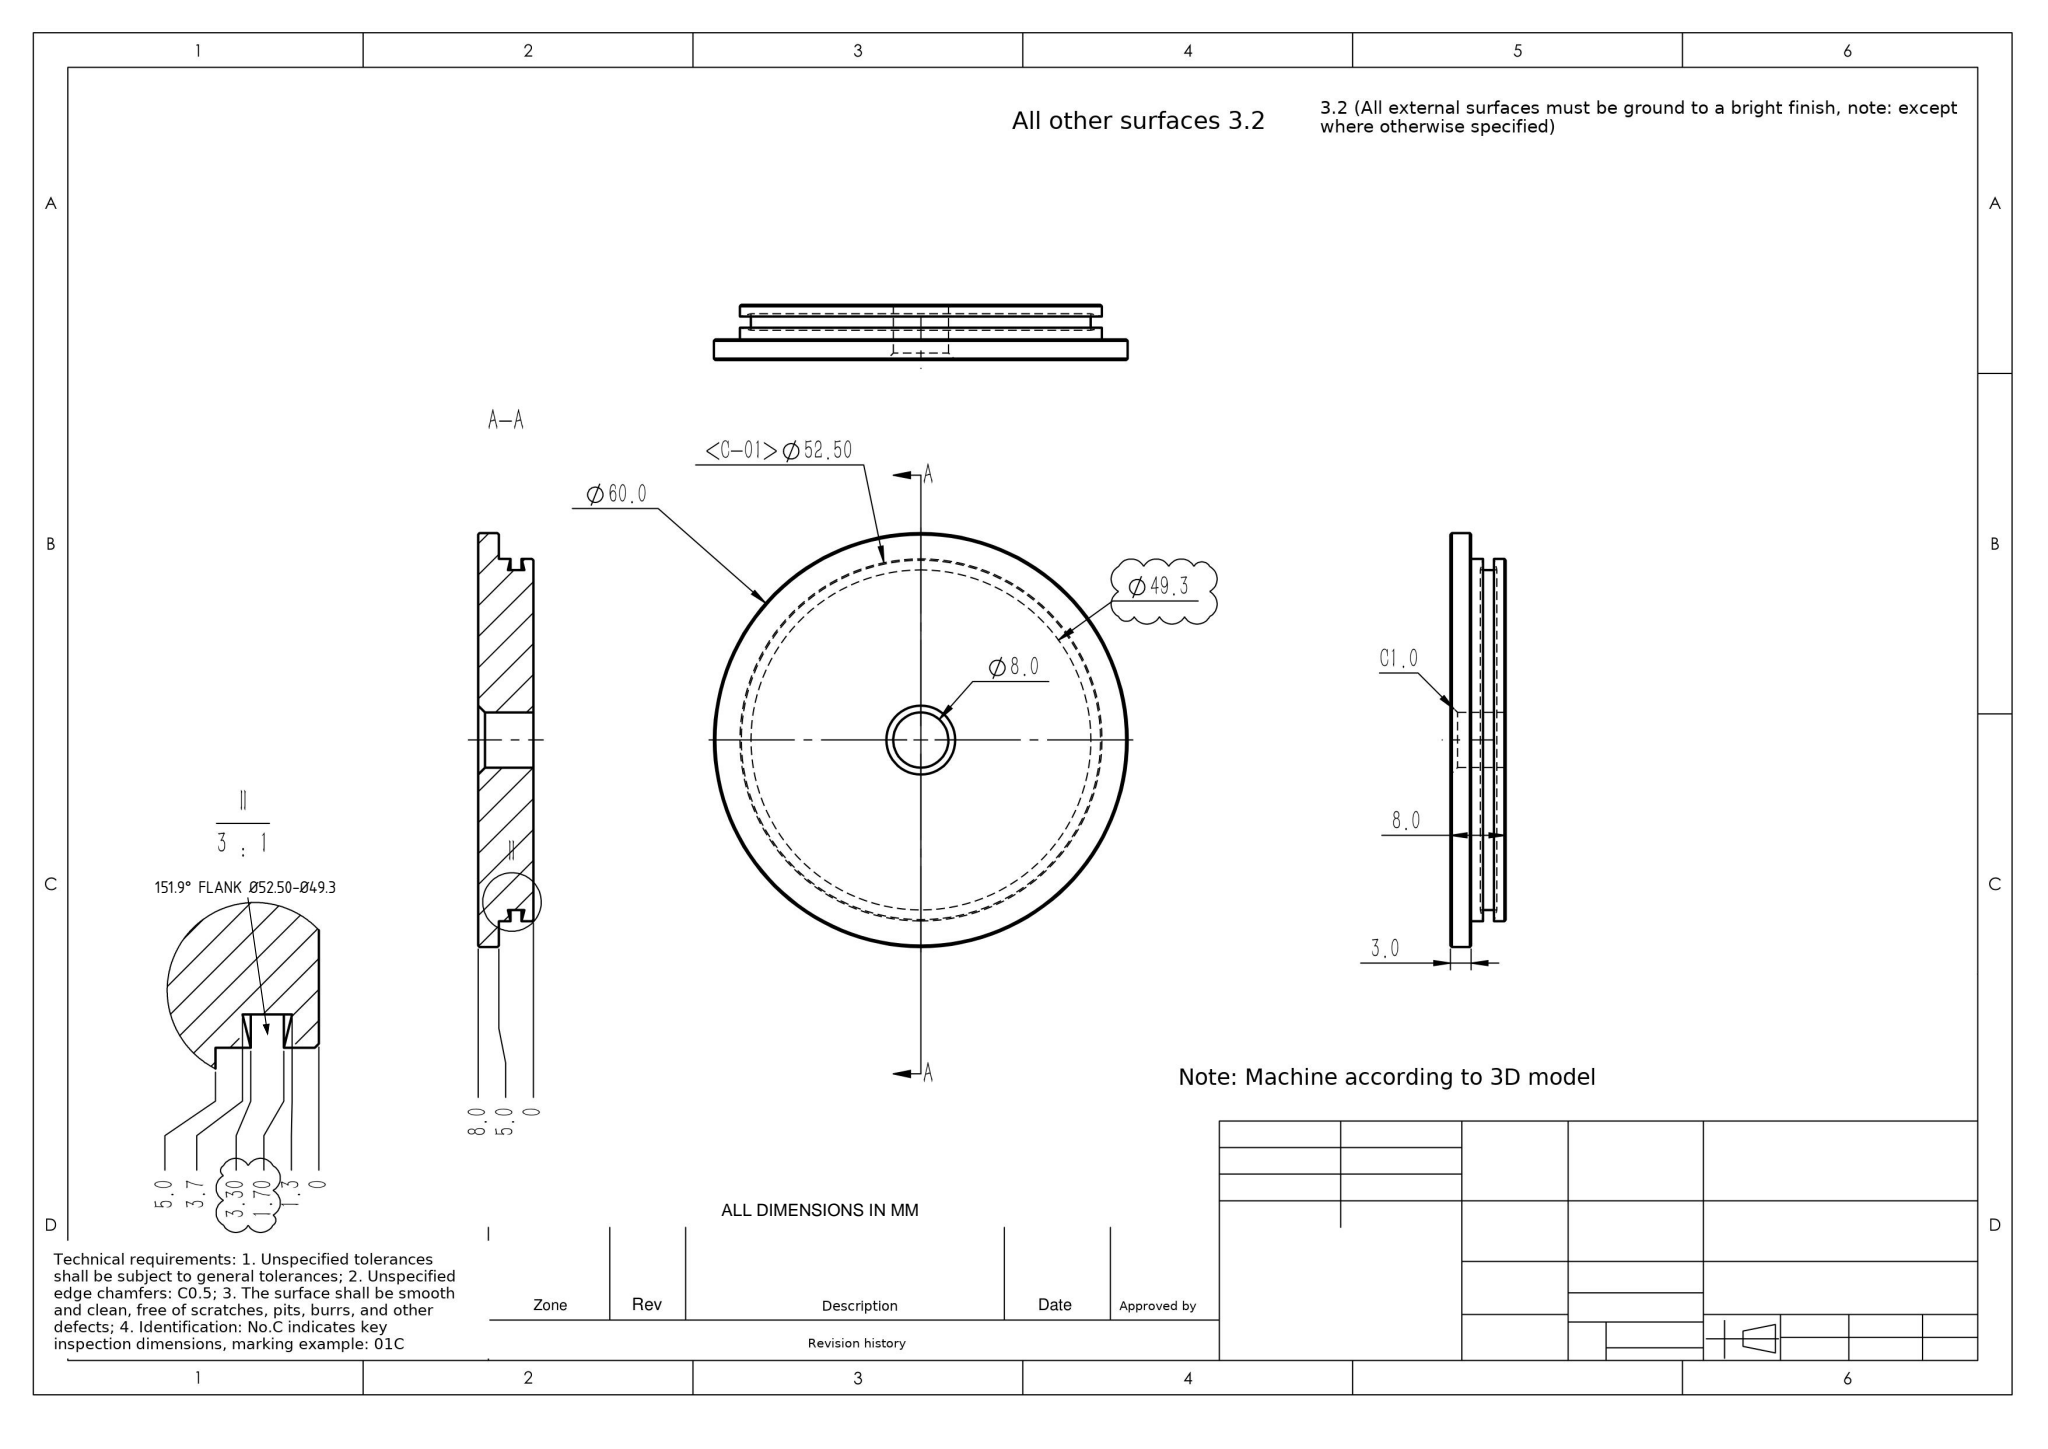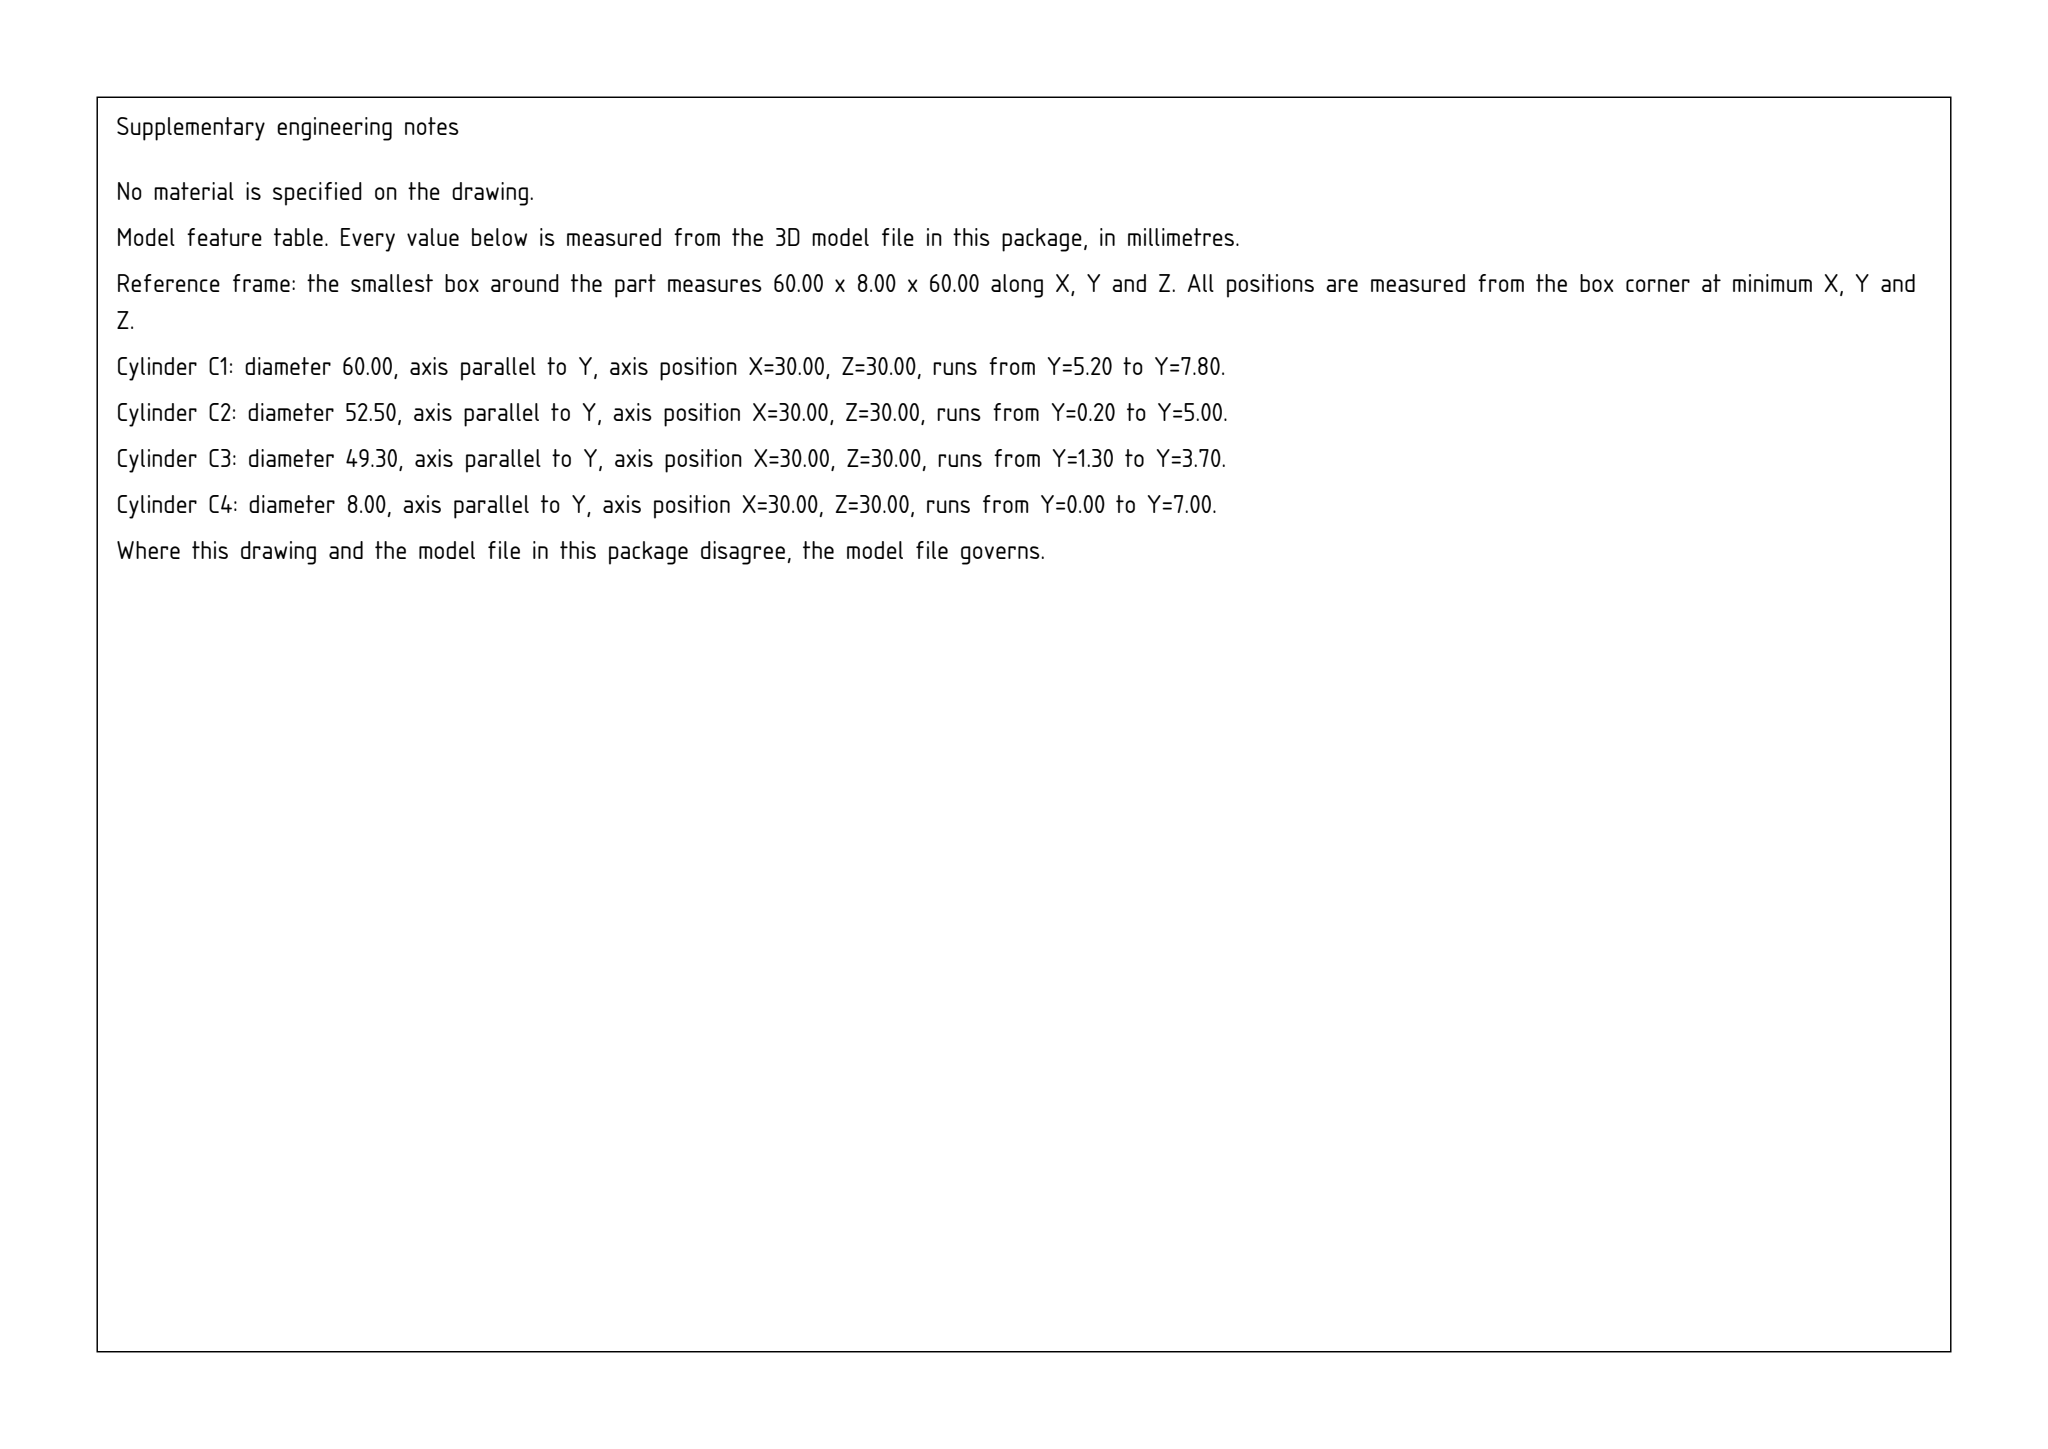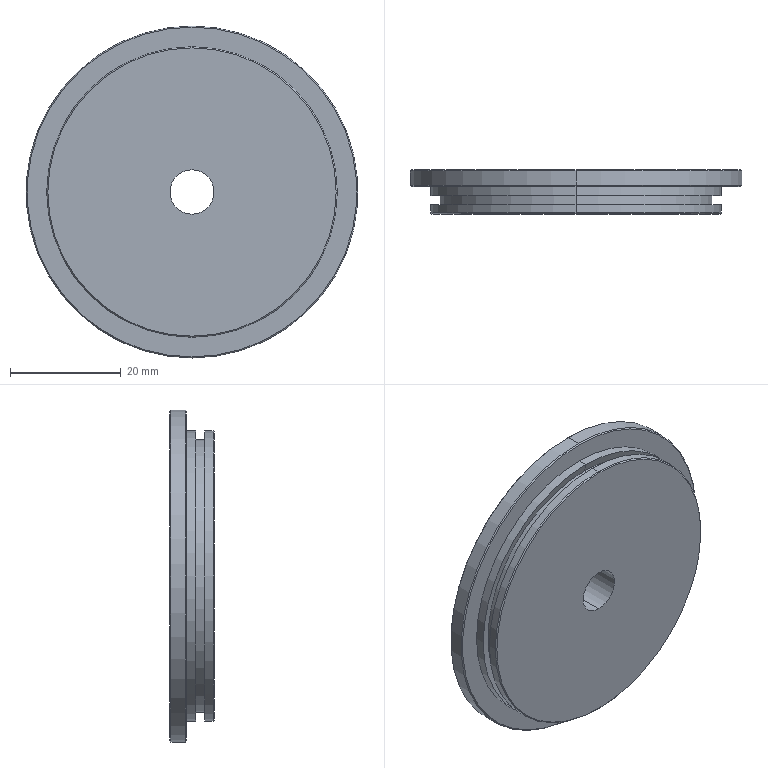Part | SolidWorks | mm | 1 solid | 25 faces | box 60 x 8 x 60 mm | volume 18369 mm3 | cone 12 | cylinder 10 | plane 3 | commonest cylinder face diameters 52.5 x4 49.3 x2 8 x2 60 x2
Drawing notes:
DETAIL II: GROOVE FLANK 151.9° INCL, Ø52.50 TO Ø49.3 | from the solid: cones[included_angle,ref_dia]: [151.9, 52.5] and [151.9, 49.3], both x2
build123d program:
from build123d import *

# Parameters (mm, degrees)
SKETCH1_R           = 30
BOSS_EXTRUDE1_DEPTH = 3
SKETCH2_R           = 4
CUT_EXTRUDE1_DEPTH  = 5
CHAMFER1_SIZE       = 1
SKETCH3_R           = 26.25
SKETCH3_R_2         = 4
BOSS_EXTRUDE2_DEPTH = 5
CHAMFER2_SIZE       = 0.2


with BuildPart() as part:
    # Sketch1 → Boss-Extrude1 (new body)
    with BuildSketch(Plane(origin=(0, 0, 0), x_dir=(1, 0, 0), z_dir=(0, 1, 0))):
        with Locations(Location((0, 0, 0), (0, 0, 270))):
            Circle(SKETCH1_R)
    extrude(amount=BOSS_EXTRUDE1_DEPTH)

    # Sketch2 → Cut-Extrude1 (cut)
    with BuildSketch(Plane(origin=(0, 3, 0), x_dir=(1, 0, 0), z_dir=(0, 1, 0))):
        with Locations(Location((0, 0, 0), (0, 0, 270))):
            Circle(SKETCH2_R)
    extrude(amount=-CUT_EXTRUDE1_DEPTH, mode=Mode.SUBTRACT)

    # Chamfer1
    chamfer1_edges = [part.edges().sort_by_distance(p)[0] for p in [
        (0, 3, -4),
    ]]
    chamfer(chamfer1_edges, length=CHAMFER1_SIZE)

    # Sketch3 → Boss-Extrude2 (add)
    with BuildSketch(Plane.XZ):
        with Locations(Location((0, 0, 0), (0, 0, 90))):
            Circle(SKETCH3_R)
        with Locations(Location((0, 0, 0), (0, 0, 90))):
            Circle(SKETCH3_R_2, mode=Mode.SUBTRACT)
    extrude(amount=BOSS_EXTRUDE2_DEPTH)

    # Sketch5 → Cut-Revolve1 (revolve, cut)
    with BuildSketch(Plane.XY, mode=Mode.PRIVATE) as cut_revolve1_sk:
        Polygon((-26.25, -1.7), (-26.25, -3.3), (-24.65, -3.7), (-24.65, -1.3), align=None)
    revolve(cut_revolve1_sk.sketch.rotate(Axis((0, -2, 0), (0, 1, 0)), 270), axis=Axis((0, -2, 0), (0, 1, 0)), mode=Mode.SUBTRACT)

    # Chamfer2
    chamfer2_edges = [part.edges().sort_by_distance(p)[0] for p in [
        (0, -5, -26.25),
        (0, 0, -30),
        (0, 3, -30),
    ]]
    chamfer(chamfer2_edges, length=CHAMFER2_SIZE)


solid = part.part
STEP:
#1=CARTESIAN_POINT('',(0.,-5.,-26.05));
#2=VERTEX_POINT('',#1);
#3=CARTESIAN_POINT('',(0.,-5.,26.05));
#4=VERTEX_POINT('',#3);
#5=CARTESIAN_POINT('',(0.,-5.,0.));
#6=DIRECTION('',(0.,-1.,0.));
#7=DIRECTION('',(0.,0.,-1.));
#8=AXIS2_PLACEMENT_3D('',#5,#6,#7);
#9=CIRCLE('',#8,26.05);
#10=EDGE_CURVE('',#2,#4,#9,.T.);
#11=ORIENTED_EDGE('',*,*,#10,.F.);
#12=CARTESIAN_POINT('',(0.,-4.8,-26.25));
#13=VERTEX_POINT('',#12);
#14=CARTESIAN_POINT('',(0.,-5.,-26.05));
#15=DIRECTION('',(0.,0.7071,-0.7071));
#16=VECTOR('',#15,1000.);
#17=LINE('',#14,#16);
#18=EDGE_CURVE('',#2,#13,#17,.T.);
#19=ORIENTED_EDGE('',*,*,#18,.T.);
#20=CARTESIAN_POINT('',(0.,-4.8,26.25));
#21=VERTEX_POINT('',#20);
#22=CARTESIAN_POINT('',(0.,-4.8,0.));
#23=DIRECTION('',(0.,1.,0.));
#24=DIRECTION('',(0.,0.,-1.));
#25=AXIS2_PLACEMENT_3D('',#22,#23,#24);
#26=CIRCLE('',#25,26.25);
#27=EDGE_CURVE('',#21,#13,#26,.T.);
#28=ORIENTED_EDGE('',*,*,#27,.F.);
#29=CARTESIAN_POINT('',(0.,-5.,26.05));
#30=DIRECTION('',(0.,0.7071,0.7071));
#31=VECTOR('',#30,1000.);
#32=LINE('',#29,#31);
#33=EDGE_CURVE('',#4,#21,#32,.T.);
#34=ORIENTED_EDGE('',*,*,#33,.F.);
#35=EDGE_LOOP('',(#11,#19,#28,#34));
#36=FACE_OUTER_BOUND('',#35,.T.);
#37=CARTESIAN_POINT('',(0.,-5.,0.));
#38=DIRECTION('',(0.,1.,0.));
#39=DIRECTION('',(0.,0.,1.));
#40=AXIS2_PLACEMENT_3D('',#37,#38,#39);
#41=CONICAL_SURFACE('',#40,26.05,0.7854);
#42=ADVANCED_FACE('',(#36),#41,.T.);
#43=CARTESIAN_POINT('',(0.,3.,29.8));
#44=VERTEX_POINT('',#43);
#45=CARTESIAN_POINT('',(0.,3.,-29.8));
#46=VERTEX_POINT('',#45);
#47=CARTESIAN_POINT('',(0.,3.,0.));
#48=DIRECTION('',(0.,1.,0.));
#49=DIRECTION('',(0.,0.,1.));
#50=AXIS2_PLACEMENT_3D('',#47,#48,#49);
#51=CIRCLE('',#50,29.8);
#52=EDGE_CURVE('',#44,#46,#51,.T.);
#53=ORIENTED_EDGE('',*,*,#52,.F.);
#54=CARTESIAN_POINT('',(0.,2.8,30.));
#55=VERTEX_POINT('',#54);
#56=CARTESIAN_POINT('',(0.,3.,29.8));
#57=DIRECTION('',(0.,-0.7071,0.7071));
#58=VECTOR('',#57,1000.);
#59=LINE('',#56,#58);
#60=EDGE_CURVE('',#44,#55,#59,.T.);
#61=ORIENTED_EDGE('',*,*,#60,.T.);
#62=CARTESIAN_POINT('',(0.,2.8,-30.));
#63=VERTEX_POINT('',#62);
#64=CARTESIAN_POINT('',(0.,2.8,0.));
#65=DIRECTION('',(0.,-1.,0.));
#66=DIRECTION('',(0.,0.,1.));
#67=AXIS2_PLACEMENT_3D('',#64,#65,#66);
#68=CIRCLE('',#67,30.);
#69=EDGE_CURVE('',#63,#55,#68,.T.);
#70=ORIENTED_EDGE('',*,*,#69,.F.);
#71=CARTESIAN_POINT('',(0.,3.,-29.8));
#72=DIRECTION('',(0.,-0.7071,-0.7071));
#73=VECTOR('',#72,1000.);
#74=LINE('',#71,#73);
#75=EDGE_CURVE('',#46,#63,#74,.T.);
#76=ORIENTED_EDGE('',*,*,#75,.F.);
#77=EDGE_LOOP('',(#53,#61,#70,#76));
#78=FACE_OUTER_BOUND('',#77,.T.);
#79=CARTESIAN_POINT('',(0.,3.,0.));
#80=DIRECTION('',(0.,-1.,0.));
#81=DIRECTION('',(0.,0.,-1.));
#82=AXIS2_PLACEMENT_3D('',#79,#80,#81);
#83=CONICAL_SURFACE('',#82,29.8,0.7854);
#84=ADVANCED_FACE('',(#78),#83,.T.);
#85=CARTESIAN_POINT('',(0.,0.,-29.8));
#86=VERTEX_POINT('',#85);
#87=CARTESIAN_POINT('',(0.,0.,29.8));
#88=VERTEX_POINT('',#87);
#89=CARTESIAN_POINT('',(0.,0.,0.));
#90=DIRECTION('',(0.,-1.,0.));
#91=DIRECTION('',(0.,0.,1.));
#92=AXIS2_PLACEMENT_3D('',#89,#90,#91);
#93=CIRCLE('',#92,29.8);
#94=EDGE_CURVE('',#86,#88,#93,.T.);
#95=ORIENTED_EDGE('',*,*,#94,.F.);
#96=CARTESIAN_POINT('',(0.,0.2,-30.));
#97=VERTEX_POINT('',#96);
#98=CARTESIAN_POINT('',(0.,0.2,-30.));
#99=DIRECTION('',(0.,0.7071,-0.7071));
#100=VECTOR('',#99,1000.);
#101=LINE('',#98,#100);
#102=EDGE_CURVE('',#86,#97,#101,.T.);
#103=ORIENTED_EDGE('',*,*,#102,.T.);
#104=CARTESIAN_POINT('',(0.,0.2,30.));
#105=VERTEX_POINT('',#104);
#106=CARTESIAN_POINT('',(0.,0.2,0.));
#107=DIRECTION('',(0.,1.,0.));
#108=DIRECTION('',(0.,0.,1.));
#109=AXIS2_PLACEMENT_3D('',#106,#107,#108);
#110=CIRCLE('',#109,30.);
#111=EDGE_CURVE('',#105,#97,#110,.T.);
#112=ORIENTED_EDGE('',*,*,#111,.F.);
#113=CARTESIAN_POINT('',(0.,0.2,30.));
#114=DIRECTION('',(0.,0.7071,0.7071));
#115=VECTOR('',#114,1000.);
#116=LINE('',#113,#115);
#117=EDGE_CURVE('',#88,#105,#116,.T.);
#118=ORIENTED_EDGE('',*,*,#117,.F.);
#119=EDGE_LOOP('',(#95,#103,#112,#118));
#120=FACE_OUTER_BOUND('',#119,.T.);
#121=CARTESIAN_POINT('',(0.,0.2,0.));
#122=DIRECTION('',(0.,1.,0.));
#123=DIRECTION('',(0.,0.,1.));
#124=AXIS2_PLACEMENT_3D('',#121,#122,#123);
#125=CONICAL_SURFACE('',#124,30.,0.7854);
#126=ADVANCED_FACE('',(#120),#125,.T.);
#127=CARTESIAN_POINT('',(0.,-3.7,24.65));
#128=VERTEX_POINT('',#127);
#129=CARTESIAN_POINT('',(0.,-3.7,-24.65));
#130=VERTEX_POINT('',#129);
#131=CARTESIAN_POINT('',(0.,-3.7,0.));
#132=DIRECTION('',(0.,-1.,0.));
#133=DIRECTION('',(0.,0.,-1.));
#134=AXIS2_PLACEMENT_3D('',#131,#132,#133);
#135=CIRCLE('',#134,24.65);
#136=EDGE_CURVE('',#128,#130,#135,.T.);
#137=ORIENTED_EDGE('',*,*,#136,.T.);
#138=CARTESIAN_POINT('',(0.,-3.3,-26.25));
#139=VERTEX_POINT('',#138);
#140=CARTESIAN_POINT('',(0.,-3.3,-26.25));
#141=DIRECTION('',(0.,0.2425,-0.9701));
#142=VECTOR('',#141,1000.);
#143=LINE('',#140,#142);
#144=EDGE_CURVE('',#130,#139,#143,.T.);
#145=ORIENTED_EDGE('',*,*,#144,.T.);
#146=CARTESIAN_POINT('',(0.,-3.3,26.25));
#147=VERTEX_POINT('',#146);
#148=CARTESIAN_POINT('',(0.,-3.3,0.));
#149=DIRECTION('',(0.,-1.,0.));
#150=DIRECTION('',(0.,0.,-1.));
#151=AXIS2_PLACEMENT_3D('',#148,#149,#150);
#152=CIRCLE('',#151,26.25);
#153=EDGE_CURVE('',#147,#139,#152,.T.);
#154=ORIENTED_EDGE('',*,*,#153,.F.);
#155=CARTESIAN_POINT('',(0.,-3.3,26.25));
#156=DIRECTION('',(0.,0.2425,0.9701));
#157=VECTOR('',#156,1000.);
#158=LINE('',#155,#157);
#159=EDGE_CURVE('',#128,#147,#158,.T.);
#160=ORIENTED_EDGE('',*,*,#159,.F.);
#161=EDGE_LOOP('',(#137,#145,#154,#160));
#162=FACE_OUTER_BOUND('',#161,.T.);
#163=CARTESIAN_POINT('',(0.,-3.3,0.));
#164=DIRECTION('',(0.,1.,0.));
#165=DIRECTION('',(0.,0.,1.));
#166=AXIS2_PLACEMENT_3D('',#163,#164,#165);
#167=CONICAL_SURFACE('',#166,26.25,1.326);
#168=ADVANCED_FACE('',(#162),#167,.F.);
#169=CARTESIAN_POINT('',(0.,-1.3,-24.65));
#170=VERTEX_POINT('',#169);
#171=CARTESIAN_POINT('',(0.,-1.3,24.65));
#172=VERTEX_POINT('',#171);
#173=CARTESIAN_POINT('',(0.,-1.3,0.));
#174=DIRECTION('',(0.,-1.,0.));
#175=DIRECTION('',(0.,0.,-1.));
#176=AXIS2_PLACEMENT_3D('',#173,#174,#175);
#177=CIRCLE('',#176,24.65);
#178=EDGE_CURVE('',#170,#172,#177,.T.);
#179=ORIENTED_EDGE('',*,*,#178,.T.);
#180=CARTESIAN_POINT('',(0.,-5.,24.65));
#181=DIRECTION('',(0.,-1.,0.));
#182=VECTOR('',#181,1000.);
#183=LINE('',#180,#182);
#184=EDGE_CURVE('',#172,#128,#183,.T.);
#185=ORIENTED_EDGE('',*,*,#184,.T.);
#186=CARTESIAN_POINT('',(0.,-3.7,0.));
#187=DIRECTION('',(0.,-1.,0.));
#188=DIRECTION('',(0.,0.,-1.));
#189=AXIS2_PLACEMENT_3D('',#186,#187,#188);
#190=CIRCLE('',#189,24.65);
#191=EDGE_CURVE('',#130,#128,#190,.T.);
#192=ORIENTED_EDGE('',*,*,#191,.F.);
#193=CARTESIAN_POINT('',(0.,-5.,-24.65));
#194=DIRECTION('',(0.,-1.,0.));
#195=VECTOR('',#194,1000.);
#196=LINE('',#193,#195);
#197=EDGE_CURVE('',#170,#130,#196,.T.);
#198=ORIENTED_EDGE('',*,*,#197,.F.);
#199=EDGE_LOOP('',(#179,#185,#192,#198));
#200=FACE_OUTER_BOUND('',#199,.T.);
#201=CARTESIAN_POINT('',(0.,-5.,0.));
#202=DIRECTION('',(0.,-1.,0.));
#203=DIRECTION('',(0.,0.,-1.));
#204=AXIS2_PLACEMENT_3D('',#201,#202,#203);
#205=CYLINDRICAL_SURFACE('',#204,24.65);
#206=ADVANCED_FACE('',(#200),#205,.T.);
#207=CARTESIAN_POINT('',(0.,-1.3,0.));
#208=DIRECTION('',(0.,-1.,0.));
#209=DIRECTION('',(0.,0.,-1.));
#210=AXIS2_PLACEMENT_3D('',#207,#208,#209);
#211=CIRCLE('',#210,24.65);
#212=EDGE_CURVE('',#172,#170,#211,.T.);
#213=ORIENTED_EDGE('',*,*,#212,.F.);
#214=CARTESIAN_POINT('',(0.,-1.7,26.25));
#215=VERTEX_POINT('',#214);
#216=CARTESIAN_POINT('',(0.,-1.3,24.65));
#217=DIRECTION('',(0.,-0.2425,0.9701));
#218=VECTOR('',#217,1000.);
#219=LINE('',#216,#218);
#220=EDGE_CURVE('',#172,#215,#219,.T.);
#221=ORIENTED_EDGE('',*,*,#220,.T.);
#222=CARTESIAN_POINT('',(0.,-1.7,-26.25));
#223=VERTEX_POINT('',#222);
#224=CARTESIAN_POINT('',(0.,-1.7,0.));
#225=DIRECTION('',(0.,-1.,0.));
#226=DIRECTION('',(0.,0.,-1.));
#227=AXIS2_PLACEMENT_3D('',#224,#225,#226);
#228=CIRCLE('',#227,26.25);
#229=EDGE_CURVE('',#215,#223,#228,.T.);
#230=ORIENTED_EDGE('',*,*,#229,.T.);
#231=CARTESIAN_POINT('',(0.,-1.3,-24.65));
#232=DIRECTION('',(0.,-0.2425,-0.9701));
#233=VECTOR('',#232,1000.);
#234=LINE('',#231,#233);
#235=EDGE_CURVE('',#170,#223,#234,.T.);
#236=ORIENTED_EDGE('',*,*,#235,.F.);
#237=EDGE_LOOP('',(#213,#221,#230,#236));
#238=FACE_OUTER_BOUND('',#237,.T.);
#239=CARTESIAN_POINT('',(0.,-1.3,0.));
#240=DIRECTION('',(0.,-1.,0.));
#241=DIRECTION('',(0.,0.,-1.));
#242=AXIS2_PLACEMENT_3D('',#239,#240,#241);
#243=CONICAL_SURFACE('',#242,24.65,1.326);
#244=ADVANCED_FACE('',(#238),#243,.F.);
#245=CARTESIAN_POINT('',(0.,2.,-4.));
#246=VERTEX_POINT('',#245);
#247=CARTESIAN_POINT('',(0.,2.,4.));
#248=VERTEX_POINT('',#247);
#249=CARTESIAN_POINT('',(0.,2.,0.));
#250=DIRECTION('',(0.,1.,0.));
#251=DIRECTION('',(0.,0.,1.));
#252=AXIS2_PLACEMENT_3D('',#249,#250,#251);
#253=CIRCLE('',#252,4.);
#254=EDGE_CURVE('',#246,#248,#253,.T.);
#255=ORIENTED_EDGE('',*,*,#254,.F.);
#256=CARTESIAN_POINT('',(0.,3.,-5.));
#257=VERTEX_POINT('',#256);
#258=CARTESIAN_POINT('',(0.,2.,-4.));
#259=DIRECTION('',(0.,0.7071,-0.7071));
#260=VECTOR('',#259,1000.);
#261=LINE('',#258,#260);
#262=EDGE_CURVE('',#246,#257,#261,.T.);
#263=ORIENTED_EDGE('',*,*,#262,.T.);
#264=CARTESIAN_POINT('',(0.,3.,5.));
#265=VERTEX_POINT('',#264);
#266=CARTESIAN_POINT('',(0.,3.,0.));
#267=DIRECTION('',(0.,-1.,0.));
#268=DIRECTION('',(0.,0.,1.));
#269=AXIS2_PLACEMENT_3D('',#266,#267,#268);
#270=CIRCLE('',#269,5.);
#271=EDGE_CURVE('',#265,#257,#270,.T.);
#272=ORIENTED_EDGE('',*,*,#271,.F.);
#273=CARTESIAN_POINT('',(0.,2.,4.));
#274=DIRECTION('',(0.,0.7071,0.7071));
#275=VECTOR('',#274,1000.);
#276=LINE('',#273,#275);
#277=EDGE_CURVE('',#248,#265,#276,.T.);
#278=ORIENTED_EDGE('',*,*,#277,.F.);
#279=EDGE_LOOP('',(#255,#263,#272,#278));
#280=FACE_OUTER_BOUND('',#279,.T.);
#281=CARTESIAN_POINT('',(0.,2.,0.));
#282=DIRECTION('',(0.,1.,0.));
#283=DIRECTION('',(0.,0.,1.));
#284=AXIS2_PLACEMENT_3D('',#281,#282,#283);
#285=CONICAL_SURFACE('',#284,4.,0.7854);
#286=ADVANCED_FACE('',(#280),#285,.F.);
#287=CARTESIAN_POINT('',(0.,-5.,4.));
#288=VERTEX_POINT('',#287);
#289=CARTESIAN_POINT('',(0.,-5.,-4.));
#290=VERTEX_POINT('',#289);
#291=CARTESIAN_POINT('',(0.,-5.,0.));
#292=DIRECTION('',(0.,-1.,0.));
#293=DIRECTION('',(0.,0.,-1.));
#294=AXIS2_PLACEMENT_3D('',#291,#292,#293);
#295=CIRCLE('',#294,4.);
#296=EDGE_CURVE('',#288,#290,#295,.T.);
#297=ORIENTED_EDGE('',*,*,#296,.T.);
#298=CARTESIAN_POINT('',(0.,-2.,-4.));
#299=DIRECTION('',(0.,1.,0.));
#300=VECTOR('',#299,1000.);
#301=LINE('',#298,#300);
#302=EDGE_CURVE('',#290,#246,#301,.T.);
#303=ORIENTED_EDGE('',*,*,#302,.T.);
#304=ORIENTED_EDGE('',*,*,#254,.T.);
#305=CARTESIAN_POINT('',(0.,-2.,4.));
#306=DIRECTION('',(0.,1.,0.));
#307=VECTOR('',#306,1000.);
#308=LINE('',#305,#307);
#309=EDGE_CURVE('',#288,#248,#308,.T.);
#310=ORIENTED_EDGE('',*,*,#309,.F.);
#311=EDGE_LOOP('',(#297,#303,#304,#310));
#312=FACE_OUTER_BOUND('',#311,.T.);
#313=CARTESIAN_POINT('',(0.,-2.,0.));
#314=DIRECTION('',(0.,1.,0.));
#315=DIRECTION('',(0.,0.,1.));
#316=AXIS2_PLACEMENT_3D('',#313,#314,#315);
#317=CYLINDRICAL_SURFACE('',#316,4.);
#318=ADVANCED_FACE('',(#312),#317,.F.);
#319=ORIENTED_EDGE('',*,*,#69,.T.);
#320=CARTESIAN_POINT('',(0.,3.,30.));
#321=DIRECTION('',(0.,-1.,0.));
#322=VECTOR('',#321,1000.);
#323=LINE('',#320,#322);
#324=EDGE_CURVE('',#55,#105,#323,.T.);
#325=ORIENTED_EDGE('',*,*,#324,.T.);
#326=ORIENTED_EDGE('',*,*,#111,.T.);
#327=CARTESIAN_POINT('',(0.,3.,-30.));
#328=DIRECTION('',(0.,-1.,0.));
#329=VECTOR('',#328,1000.);
#330=LINE('',#327,#329);
#331=EDGE_CURVE('',#63,#97,#330,.T.);
#332=ORIENTED_EDGE('',*,*,#331,.F.);
#333=EDGE_LOOP('',(#319,#325,#326,#332));
#334=FACE_OUTER_BOUND('',#333,.T.);
#335=CARTESIAN_POINT('',(0.,3.,0.));
#336=DIRECTION('',(0.,-1.,0.));
#337=DIRECTION('',(0.,0.,-1.));
#338=AXIS2_PLACEMENT_3D('',#335,#336,#337);
#339=CYLINDRICAL_SURFACE('',#338,30.);
#340=ADVANCED_FACE('',(#334),#339,.T.);
#341=ORIENTED_EDGE('',*,*,#27,.T.);
#342=CARTESIAN_POINT('',(0.,-5.,-26.25));
#343=DIRECTION('',(0.,1.,0.));
#344=VECTOR('',#343,1000.);
#345=LINE('',#342,#344);
#346=EDGE_CURVE('',#13,#139,#345,.T.);
#347=ORIENTED_EDGE('',*,*,#346,.T.);
#348=CARTESIAN_POINT('',(0.,-3.3,0.));
#349=DIRECTION('',(0.,-1.,0.));
#350=DIRECTION('',(0.,0.,-1.));
#351=AXIS2_PLACEMENT_3D('',#348,#349,#350);
#352=CIRCLE('',#351,26.25);
#353=EDGE_CURVE('',#139,#147,#352,.T.);
#354=ORIENTED_EDGE('',*,*,#353,.T.);
#355=CARTESIAN_POINT('',(0.,-5.,26.25));
#356=DIRECTION('',(0.,1.,0.));
#357=VECTOR('',#356,1000.);
#358=LINE('',#355,#357);
#359=EDGE_CURVE('',#21,#147,#358,.T.);
#360=ORIENTED_EDGE('',*,*,#359,.F.);
#361=EDGE_LOOP('',(#341,#347,#354,#360));
#362=FACE_OUTER_BOUND('',#361,.T.);
#363=CARTESIAN_POINT('',(0.,-5.,0.));
#364=DIRECTION('',(0.,1.,0.));
#365=DIRECTION('',(0.,0.,1.));
#366=AXIS2_PLACEMENT_3D('',#363,#364,#365);
#367=CYLINDRICAL_SURFACE('',#366,26.25);
#368=ADVANCED_FACE('',(#362),#367,.T.);
#369=CARTESIAN_POINT('',(0.,-1.7,0.));
#370=DIRECTION('',(0.,-1.,0.));
#371=DIRECTION('',(0.,0.,-1.));
#372=AXIS2_PLACEMENT_3D('',#369,#370,#371);
#373=CIRCLE('',#372,26.25);
#374=EDGE_CURVE('',#223,#215,#373,.T.);
#375=ORIENTED_EDGE('',*,*,#374,.F.);
#376=CARTESIAN_POINT('',(0.,0.,-26.25));
#377=VERTEX_POINT('',#376);
#378=CARTESIAN_POINT('',(0.,-5.,-26.25));
#379=DIRECTION('',(0.,1.,0.));
#380=VECTOR('',#379,1000.);
#381=LINE('',#378,#380);
#382=EDGE_CURVE('',#223,#377,#381,.T.);
#383=ORIENTED_EDGE('',*,*,#382,.T.);
#384=CARTESIAN_POINT('',(0.,0.,26.25));
#385=VERTEX_POINT('',#384);
#386=CARTESIAN_POINT('',(0.,0.,0.));
#387=DIRECTION('',(0.,-1.,0.));
#388=DIRECTION('',(0.,0.,1.));
#389=AXIS2_PLACEMENT_3D('',#386,#387,#388);
#390=CIRCLE('',#389,26.25);
#391=EDGE_CURVE('',#377,#385,#390,.T.);
#392=ORIENTED_EDGE('',*,*,#391,.T.);
#393=CARTESIAN_POINT('',(0.,-5.,26.25));
#394=DIRECTION('',(0.,1.,0.));
#395=VECTOR('',#394,1000.);
#396=LINE('',#393,#395);
#397=EDGE_CURVE('',#215,#385,#396,.T.);
#398=ORIENTED_EDGE('',*,*,#397,.F.);
#399=EDGE_LOOP('',(#375,#383,#392,#398));
#400=FACE_OUTER_BOUND('',#399,.T.);
#401=CARTESIAN_POINT('',(0.,-5.,0.));
#402=DIRECTION('',(0.,1.,0.));
#403=DIRECTION('',(0.,0.,1.));
#404=AXIS2_PLACEMENT_3D('',#401,#402,#403);
#405=CYLINDRICAL_SURFACE('',#404,26.25);
#406=ADVANCED_FACE('',(#400),#405,.T.);
#407=ORIENTED_EDGE('',*,*,#382,.F.);
#408=ORIENTED_EDGE('',*,*,#229,.F.);
#409=ORIENTED_EDGE('',*,*,#397,.T.);
#410=CARTESIAN_POINT('',(0.,0.,0.));
#411=DIRECTION('',(0.,-1.,0.));
#412=DIRECTION('',(0.,0.,1.));
#413=AXIS2_PLACEMENT_3D('',#410,#411,#412);
#414=CIRCLE('',#413,26.25);
#415=EDGE_CURVE('',#385,#377,#414,.T.);
#416=ORIENTED_EDGE('',*,*,#415,.T.);
#417=EDGE_LOOP('',(#407,#408,#409,#416));
#418=FACE_OUTER_BOUND('',#417,.T.);
#419=CARTESIAN_POINT('',(0.,-5.,0.));
#420=DIRECTION('',(0.,1.,0.));
#421=DIRECTION('',(0.,0.,1.));
#422=AXIS2_PLACEMENT_3D('',#419,#420,#421);
#423=CYLINDRICAL_SURFACE('',#422,26.25);
#424=ADVANCED_FACE('',(#418),#423,.T.);
#425=ORIENTED_EDGE('',*,*,#346,.F.);
#426=CARTESIAN_POINT('',(0.,-4.8,0.));
#427=DIRECTION('',(0.,1.,0.));
#428=DIRECTION('',(0.,0.,-1.));
#429=AXIS2_PLACEMENT_3D('',#426,#427,#428);
#430=CIRCLE('',#429,26.25);
#431=EDGE_CURVE('',#13,#21,#430,.T.);
#432=ORIENTED_EDGE('',*,*,#431,.T.);
#433=ORIENTED_EDGE('',*,*,#359,.T.);
#434=ORIENTED_EDGE('',*,*,#153,.T.);
#435=EDGE_LOOP('',(#425,#432,#433,#434));
#436=FACE_OUTER_BOUND('',#435,.T.);
#437=CARTESIAN_POINT('',(0.,-5.,0.));
#438=DIRECTION('',(0.,1.,0.));
#439=DIRECTION('',(0.,0.,1.));
#440=AXIS2_PLACEMENT_3D('',#437,#438,#439);
#441=CYLINDRICAL_SURFACE('',#440,26.25);
#442=ADVANCED_FACE('',(#436),#441,.T.);
#443=CARTESIAN_POINT('',(0.,0.,0.));
#444=DIRECTION('',(0.,-1.,0.));
#445=DIRECTION('',(0.,0.,1.));
#446=AXIS2_PLACEMENT_3D('',#443,#444,#445);
#447=CIRCLE('',#446,29.8);
#448=EDGE_CURVE('',#88,#86,#447,.T.);
#449=ORIENTED_EDGE('',*,*,#448,.T.);
#450=ORIENTED_EDGE('',*,*,#94,.T.);
#451=EDGE_LOOP('',(#449,#450));
#452=FACE_OUTER_BOUND('',#451,.T.);
#453=ORIENTED_EDGE('',*,*,#415,.F.);
#454=ORIENTED_EDGE('',*,*,#391,.F.);
#455=EDGE_LOOP('',(#453,#454));
#456=FACE_BOUND('',#455,.T.);
#457=CARTESIAN_POINT('',(0.,0.,0.));
#458=DIRECTION('',(0.,1.,0.));
#459=DIRECTION('',(0.,0.,1.));
#460=AXIS2_PLACEMENT_3D('',#457,#458,#459);
#461=PLANE('',#460);
#462=ADVANCED_FACE('',(#452,#456),#461,.F.);
#463=ORIENTED_EDGE('',*,*,#324,.F.);
#464=CARTESIAN_POINT('',(0.,2.8,0.));
#465=DIRECTION('',(0.,-1.,0.));
#466=DIRECTION('',(0.,0.,1.));
#467=AXIS2_PLACEMENT_3D('',#464,#465,#466);
#468=CIRCLE('',#467,30.);
#469=EDGE_CURVE('',#55,#63,#468,.T.);
#470=ORIENTED_EDGE('',*,*,#469,.T.);
#471=ORIENTED_EDGE('',*,*,#331,.T.);
#472=CARTESIAN_POINT('',(0.,0.2,0.));
#473=DIRECTION('',(0.,1.,0.));
#474=DIRECTION('',(0.,0.,1.));
#475=AXIS2_PLACEMENT_3D('',#472,#473,#474);
#476=CIRCLE('',#475,30.);
#477=EDGE_CURVE('',#97,#105,#476,.T.);
#478=ORIENTED_EDGE('',*,*,#477,.T.);
#479=EDGE_LOOP('',(#463,#470,#471,#478));
#480=FACE_OUTER_BOUND('',#479,.T.);
#481=CARTESIAN_POINT('',(0.,3.,0.));
#482=DIRECTION('',(0.,-1.,0.));
#483=DIRECTION('',(0.,0.,-1.));
#484=AXIS2_PLACEMENT_3D('',#481,#482,#483);
#485=CYLINDRICAL_SURFACE('',#484,30.);
#486=ADVANCED_FACE('',(#480),#485,.T.);
#487=CARTESIAN_POINT('',(0.,3.,0.));
#488=DIRECTION('',(0.,1.,0.));
#489=DIRECTION('',(0.,0.,1.));
#490=AXIS2_PLACEMENT_3D('',#487,#488,#489);
#491=CIRCLE('',#490,29.8);
#492=EDGE_CURVE('',#46,#44,#491,.T.);
#493=ORIENTED_EDGE('',*,*,#492,.T.);
#494=ORIENTED_EDGE('',*,*,#52,.T.);
#495=EDGE_LOOP('',(#493,#494));
#496=FACE_OUTER_BOUND('',#495,.T.);
#497=ORIENTED_EDGE('',*,*,#271,.T.);
#498=CARTESIAN_POINT('',(0.,3.,0.));
#499=DIRECTION('',(0.,-1.,0.));
#500=DIRECTION('',(0.,0.,1.));
#501=AXIS2_PLACEMENT_3D('',#498,#499,#500);
#502=CIRCLE('',#501,5.);
#503=EDGE_CURVE('',#257,#265,#502,.T.);
#504=ORIENTED_EDGE('',*,*,#503,.T.);
#505=EDGE_LOOP('',(#497,#504));
#506=FACE_BOUND('',#505,.T.);
#507=CARTESIAN_POINT('',(0.,3.,0.));
#508=DIRECTION('',(0.,1.,0.));
#509=DIRECTION('',(0.,0.,1.));
#510=AXIS2_PLACEMENT_3D('',#507,#508,#509);
#511=PLANE('',#510);
#512=ADVANCED_FACE('',(#496,#506),#511,.T.);
#513=ORIENTED_EDGE('',*,*,#302,.F.);
#514=CARTESIAN_POINT('',(0.,-5.,0.));
#515=DIRECTION('',(0.,-1.,0.));
#516=DIRECTION('',(0.,0.,-1.));
#517=AXIS2_PLACEMENT_3D('',#514,#515,#516);
#518=CIRCLE('',#517,4.);
#519=EDGE_CURVE('',#290,#288,#518,.T.);
#520=ORIENTED_EDGE('',*,*,#519,.T.);
#521=ORIENTED_EDGE('',*,*,#309,.T.);
#522=CARTESIAN_POINT('',(0.,2.,0.));
#523=DIRECTION('',(0.,1.,0.));
#524=DIRECTION('',(0.,0.,1.));
#525=AXIS2_PLACEMENT_3D('',#522,#523,#524);
#526=CIRCLE('',#525,4.);
#527=EDGE_CURVE('',#248,#246,#526,.T.);
#528=ORIENTED_EDGE('',*,*,#527,.T.);
#529=EDGE_LOOP('',(#513,#520,#521,#528));
#530=FACE_OUTER_BOUND('',#529,.T.);
#531=CARTESIAN_POINT('',(0.,-2.,0.));
#532=DIRECTION('',(0.,1.,0.));
#533=DIRECTION('',(0.,0.,1.));
#534=AXIS2_PLACEMENT_3D('',#531,#532,#533);
#535=CYLINDRICAL_SURFACE('',#534,4.);
#536=ADVANCED_FACE('',(#530),#535,.F.);
#537=ORIENTED_EDGE('',*,*,#262,.F.);
#538=ORIENTED_EDGE('',*,*,#527,.F.);
#539=ORIENTED_EDGE('',*,*,#277,.T.);
#540=ORIENTED_EDGE('',*,*,#503,.F.);
#541=EDGE_LOOP('',(#537,#538,#539,#540));
#542=FACE_OUTER_BOUND('',#541,.T.);
#543=CARTESIAN_POINT('',(0.,2.,0.));
#544=DIRECTION('',(0.,1.,0.));
#545=DIRECTION('',(0.,0.,1.));
#546=AXIS2_PLACEMENT_3D('',#543,#544,#545);
#547=CONICAL_SURFACE('',#546,4.,0.7854);
#548=ADVANCED_FACE('',(#542),#547,.F.);
#549=CARTESIAN_POINT('',(0.,-5.,0.));
#550=DIRECTION('',(0.,-1.,0.));
#551=DIRECTION('',(0.,0.,-1.));
#552=AXIS2_PLACEMENT_3D('',#549,#550,#551);
#553=CIRCLE('',#552,26.05);
#554=EDGE_CURVE('',#4,#2,#553,.T.);
#555=ORIENTED_EDGE('',*,*,#554,.T.);
#556=ORIENTED_EDGE('',*,*,#10,.T.);
#557=EDGE_LOOP('',(#555,#556));
#558=FACE_OUTER_BOUND('',#557,.T.);
#559=ORIENTED_EDGE('',*,*,#296,.F.);
#560=ORIENTED_EDGE('',*,*,#519,.F.);
#561=EDGE_LOOP('',(#559,#560));
#562=FACE_BOUND('',#561,.T.);
#563=CARTESIAN_POINT('',(0.,-5.,0.));
#564=DIRECTION('',(0.,-1.,0.));
#565=DIRECTION('',(0.,0.,-1.));
#566=AXIS2_PLACEMENT_3D('',#563,#564,#565);
#567=PLANE('',#566);
#568=ADVANCED_FACE('',(#558,#562),#567,.T.);
#569=ORIENTED_EDGE('',*,*,#220,.F.);
#570=ORIENTED_EDGE('',*,*,#178,.F.);
#571=ORIENTED_EDGE('',*,*,#235,.T.);
#572=ORIENTED_EDGE('',*,*,#374,.T.);
#573=EDGE_LOOP('',(#569,#570,#571,#572));
#574=FACE_OUTER_BOUND('',#573,.T.);
#575=CARTESIAN_POINT('',(0.,-1.3,0.));
#576=DIRECTION('',(0.,-1.,0.));
#577=DIRECTION('',(0.,0.,-1.));
#578=AXIS2_PLACEMENT_3D('',#575,#576,#577);
#579=CONICAL_SURFACE('',#578,24.65,1.326);
#580=ADVANCED_FACE('',(#574),#579,.F.);
#581=ORIENTED_EDGE('',*,*,#184,.F.);
#582=ORIENTED_EDGE('',*,*,#212,.T.);
#583=ORIENTED_EDGE('',*,*,#197,.T.);
#584=ORIENTED_EDGE('',*,*,#136,.F.);
#585=EDGE_LOOP('',(#581,#582,#583,#584));
#586=FACE_OUTER_BOUND('',#585,.T.);
#587=CARTESIAN_POINT('',(0.,-5.,0.));
#588=DIRECTION('',(0.,-1.,0.));
#589=DIRECTION('',(0.,0.,-1.));
#590=AXIS2_PLACEMENT_3D('',#587,#588,#589);
#591=CYLINDRICAL_SURFACE('',#590,24.65);
#592=ADVANCED_FACE('',(#586),#591,.T.);
#593=ORIENTED_EDGE('',*,*,#144,.F.);
#594=ORIENTED_EDGE('',*,*,#191,.T.);
#595=ORIENTED_EDGE('',*,*,#159,.T.);
#596=ORIENTED_EDGE('',*,*,#353,.F.);
#597=EDGE_LOOP('',(#593,#594,#595,#596));
#598=FACE_OUTER_BOUND('',#597,.T.);
#599=CARTESIAN_POINT('',(0.,-3.3,0.));
#600=DIRECTION('',(0.,1.,0.));
#601=DIRECTION('',(0.,0.,1.));
#602=AXIS2_PLACEMENT_3D('',#599,#600,#601);
#603=CONICAL_SURFACE('',#602,26.25,1.326);
#604=ADVANCED_FACE('',(#598),#603,.F.);
#605=ORIENTED_EDGE('',*,*,#102,.F.);
#606=ORIENTED_EDGE('',*,*,#448,.F.);
#607=ORIENTED_EDGE('',*,*,#117,.T.);
#608=ORIENTED_EDGE('',*,*,#477,.F.);
#609=EDGE_LOOP('',(#605,#606,#607,#608));
#610=FACE_OUTER_BOUND('',#609,.T.);
#611=CARTESIAN_POINT('',(0.,0.2,0.));
#612=DIRECTION('',(0.,1.,0.));
#613=DIRECTION('',(0.,0.,1.));
#614=AXIS2_PLACEMENT_3D('',#611,#612,#613);
#615=CONICAL_SURFACE('',#614,30.,0.7854);
#616=ADVANCED_FACE('',(#610),#615,.T.);
#617=ORIENTED_EDGE('',*,*,#60,.F.);
#618=ORIENTED_EDGE('',*,*,#492,.F.);
#619=ORIENTED_EDGE('',*,*,#75,.T.);
#620=ORIENTED_EDGE('',*,*,#469,.F.);
#621=EDGE_LOOP('',(#617,#618,#619,#620));
#622=FACE_OUTER_BOUND('',#621,.T.);
#623=CARTESIAN_POINT('',(0.,3.,0.));
#624=DIRECTION('',(0.,-1.,0.));
#625=DIRECTION('',(0.,0.,-1.));
#626=AXIS2_PLACEMENT_3D('',#623,#624,#625);
#627=CONICAL_SURFACE('',#626,29.8,0.7854);
#628=ADVANCED_FACE('',(#622),#627,.T.);
#629=ORIENTED_EDGE('',*,*,#18,.F.);
#630=ORIENTED_EDGE('',*,*,#554,.F.);
#631=ORIENTED_EDGE('',*,*,#33,.T.);
#632=ORIENTED_EDGE('',*,*,#431,.F.);
#633=EDGE_LOOP('',(#629,#630,#631,#632));
#634=FACE_OUTER_BOUND('',#633,.T.);
#635=CARTESIAN_POINT('',(0.,-5.,0.));
#636=DIRECTION('',(0.,1.,0.));
#637=DIRECTION('',(0.,0.,1.));
#638=AXIS2_PLACEMENT_3D('',#635,#636,#637);
#639=CONICAL_SURFACE('',#638,26.05,0.7854);
#640=ADVANCED_FACE('',(#634),#639,.T.);
#641=CLOSED_SHELL('',(#42,#84,#126,#168,#206,#244,#286,#318,#340,#368,#406,#424,#442,#462,#486,#512,#536,#548,#568,#580,#592,#604,#616,#628,#640));
#642=MANIFOLD_SOLID_BREP('',#641);
#643=CARTESIAN_POINT('',(0.,0.,0.));
#644=DIRECTION('',(0.,0.,1.));
#645=DIRECTION('',(1.,0.,0.));
#646=AXIS2_PLACEMENT_3D('',#643,#644,#645);
#647=(LENGTH_UNIT()NAMED_UNIT(*)SI_UNIT(.MILLI.,.METRE.));
#648=UNCERTAINTY_MEASURE_WITH_UNIT(LENGTH_MEASURE(0.00001),#647,'','');
#649=(NAMED_UNIT(*)PLANE_ANGLE_UNIT()SI_UNIT($,.RADIAN.));
#650=(NAMED_UNIT(*)SI_UNIT($,.STERADIAN.)SOLID_ANGLE_UNIT());
#651=(GEOMETRIC_REPRESENTATION_CONTEXT(3)GLOBAL_UNCERTAINTY_ASSIGNED_CONTEXT((#648))GLOBAL_UNIT_ASSIGNED_CONTEXT((#647,#649,#650))REPRESENTATION_CONTEXT('',''));
#652=ADVANCED_BREP_SHAPE_REPRESENTATION('',(#642,#646),#651);